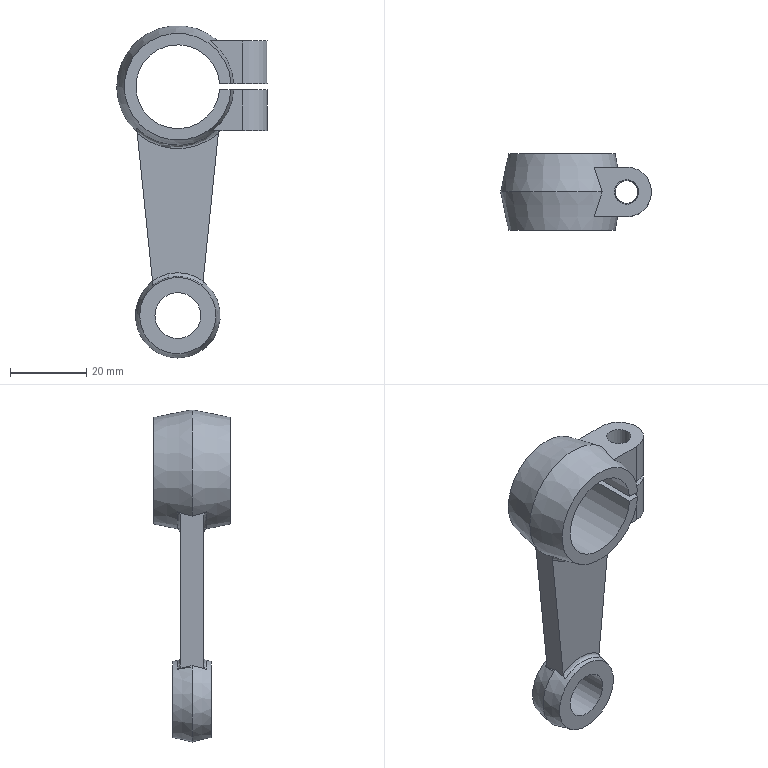Component | NX | LEVER | 1 solid | 38 faces | volume 14130 mm3 | plane 17 | cone 8 | cylinder 7 | torus 4 | spline 2 | commonest cylinder face diameters 13 x2 6 x1 22 x1 12 x1 6.4 x1 8 x1